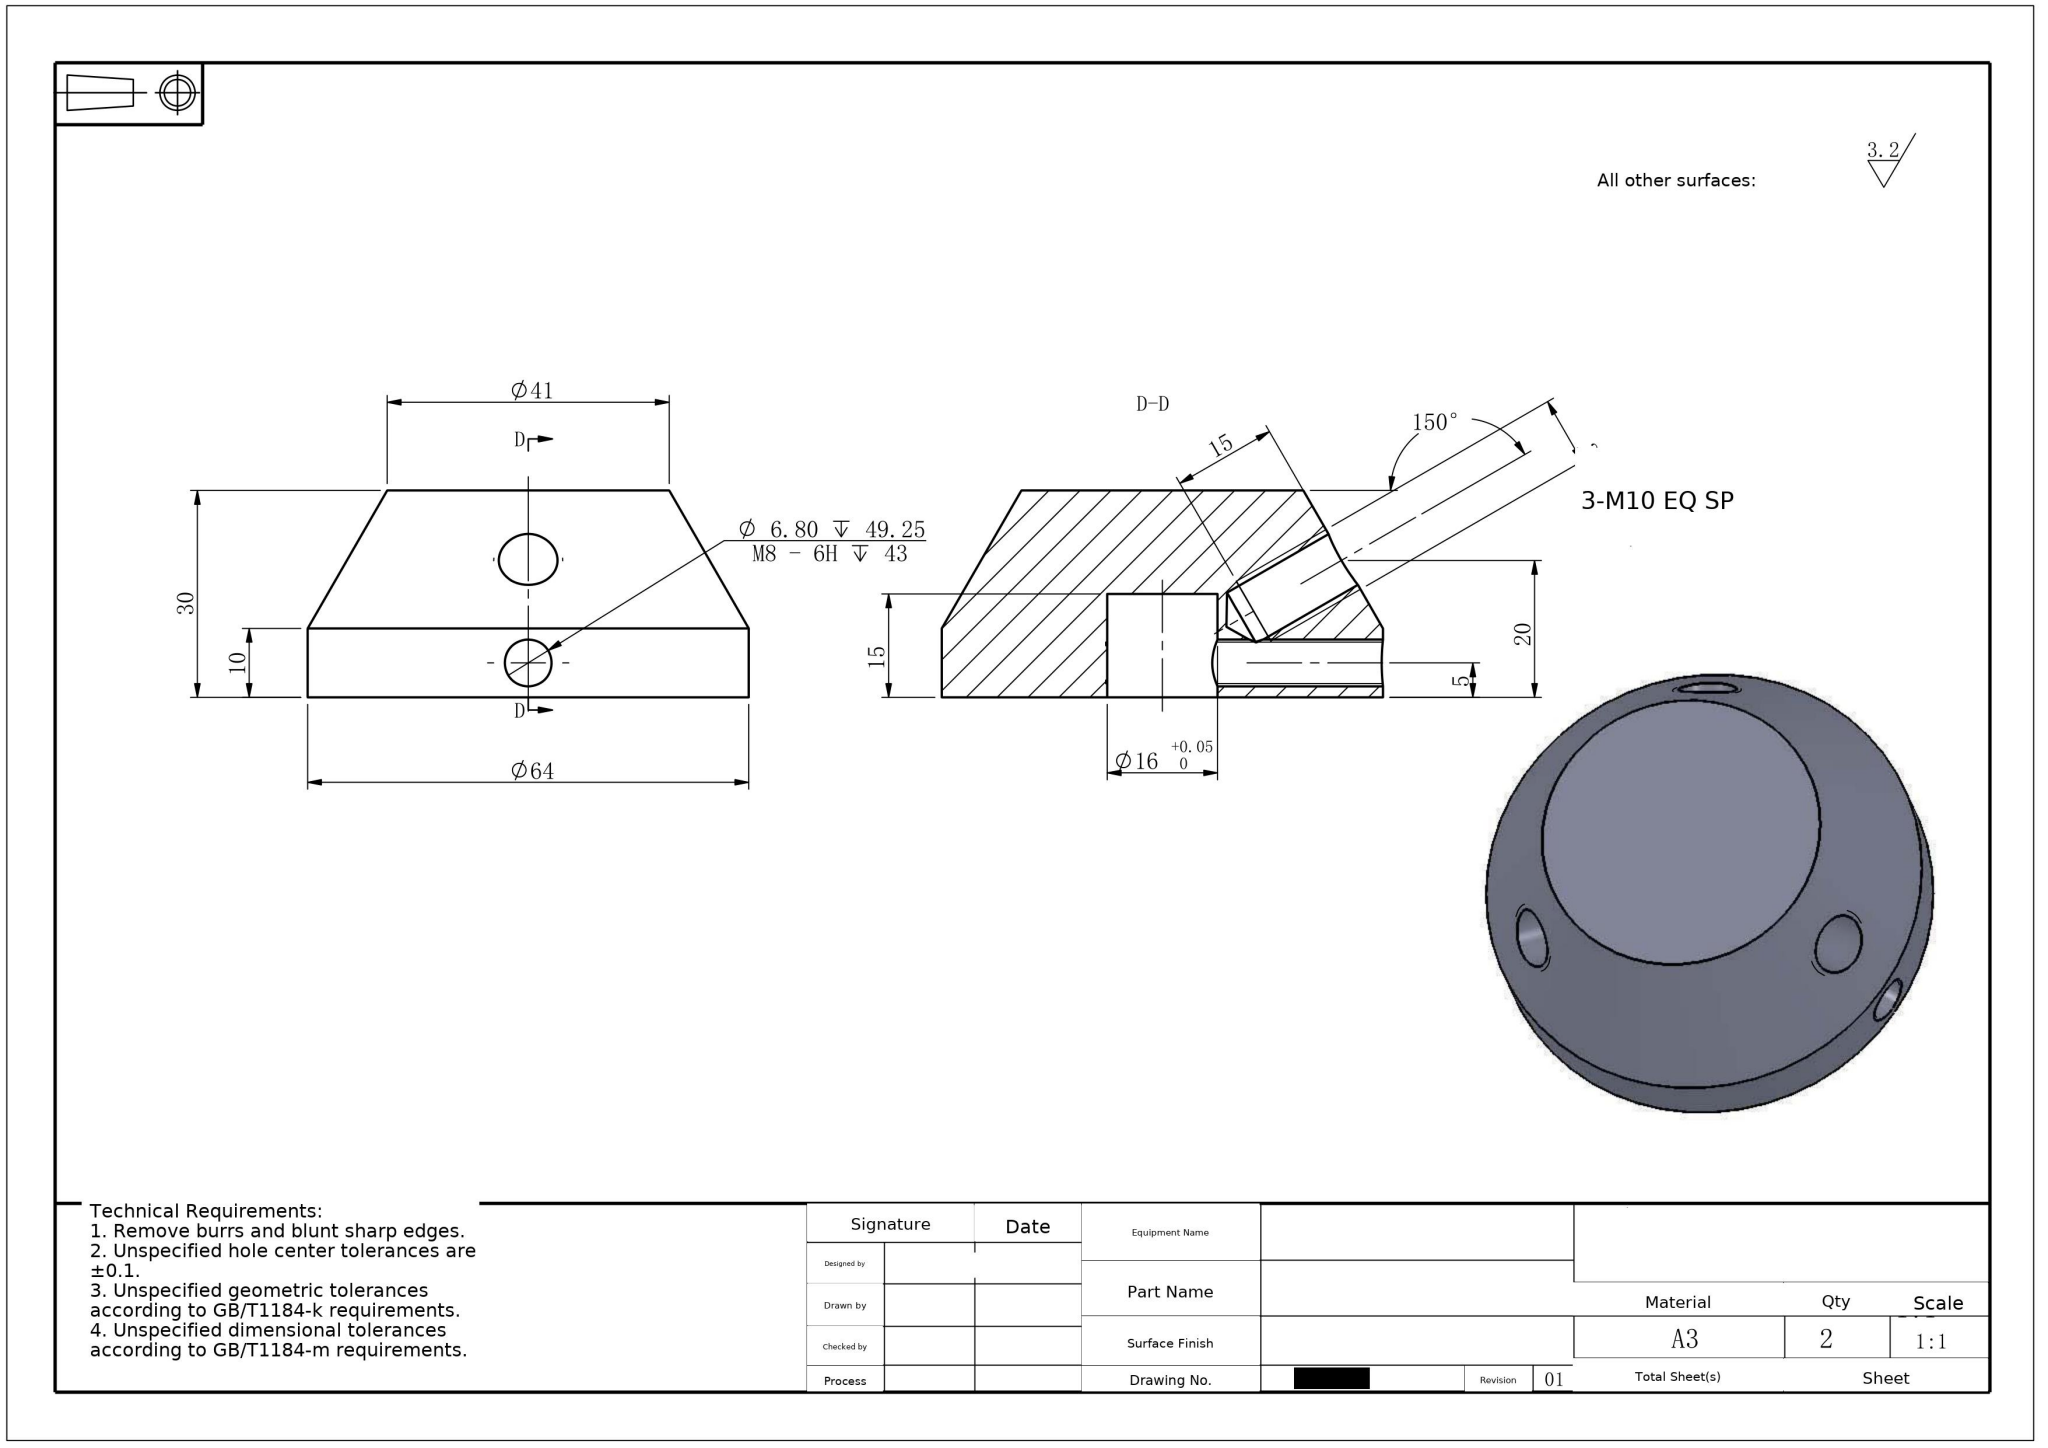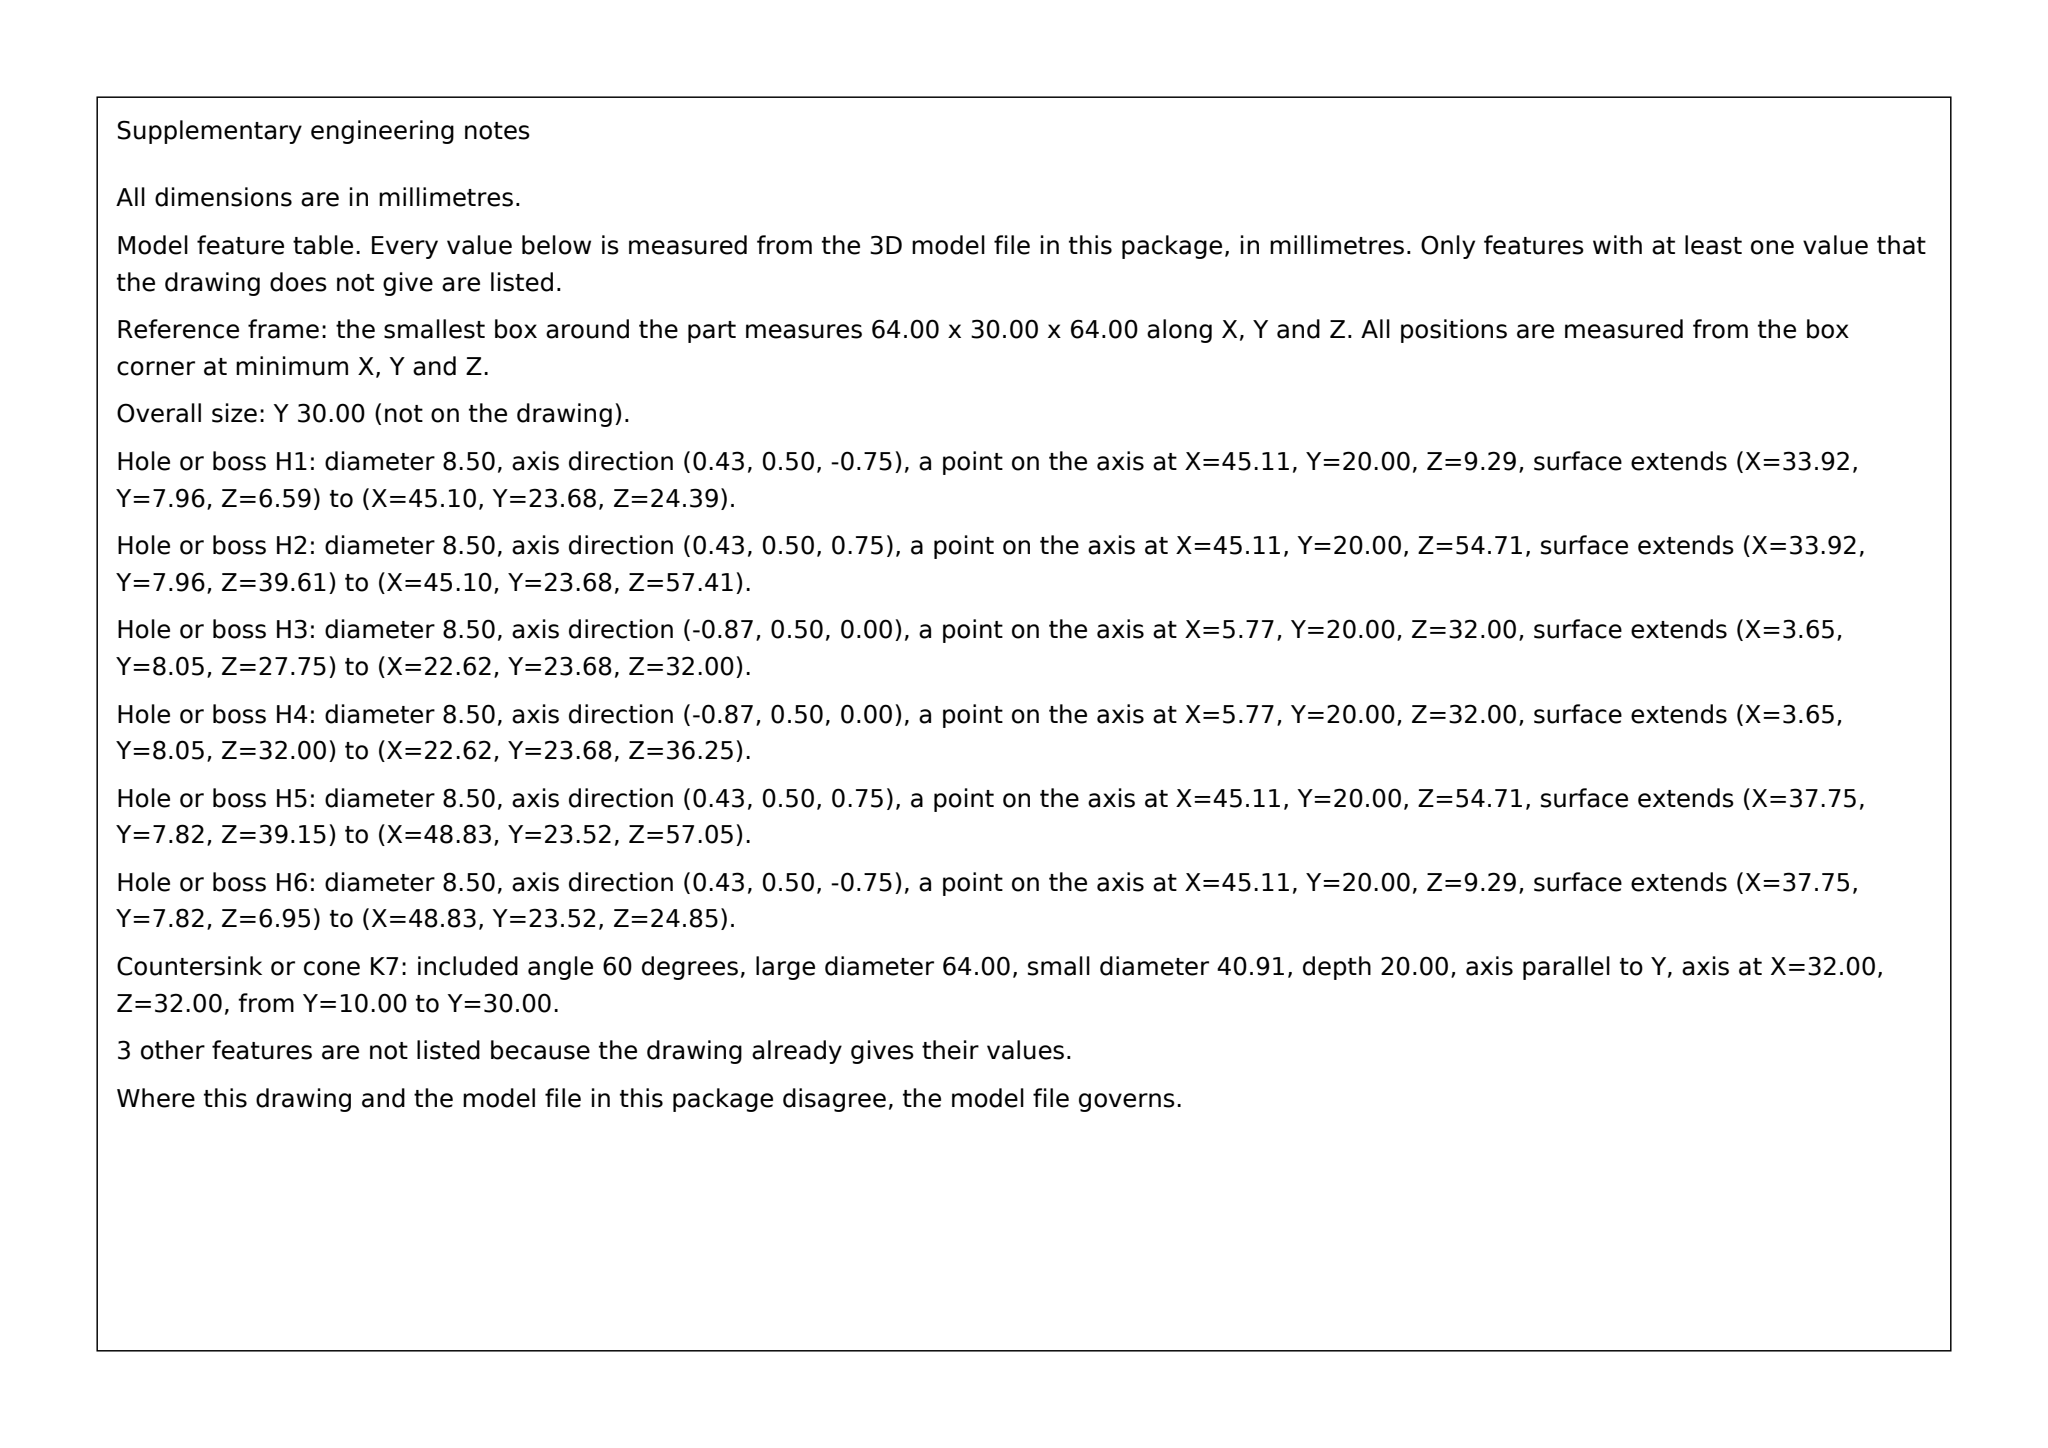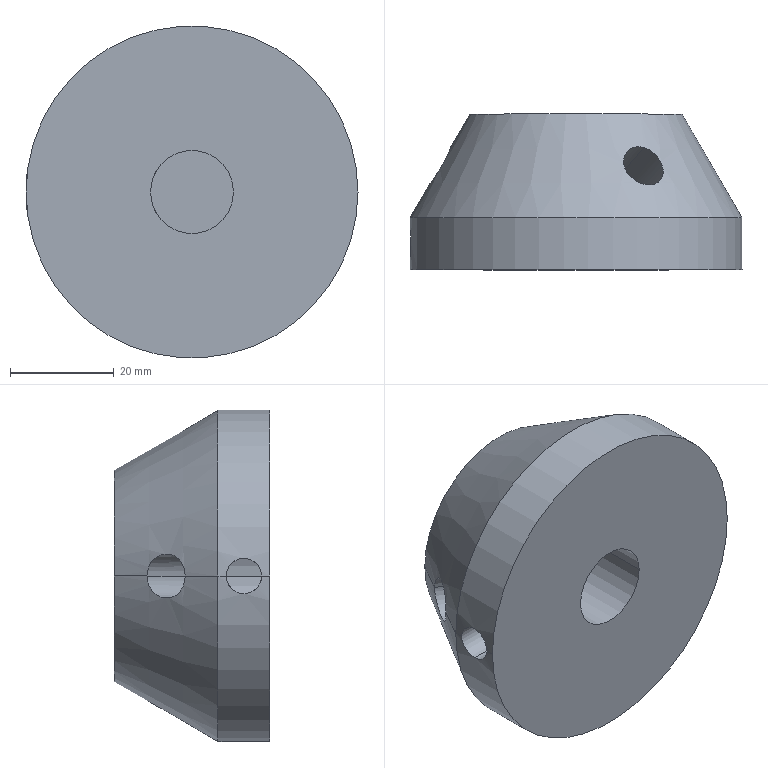Part | SolidWorks | mm | material A3 | 1 solid | 23 faces | box 64 x 30 x 64 mm | volume 69168 mm3 | cylinder 12 | cone 8 | plane 3 | commonest cylinder face diameters 8.5 x6 6.8 x2 16 x2 64 x2